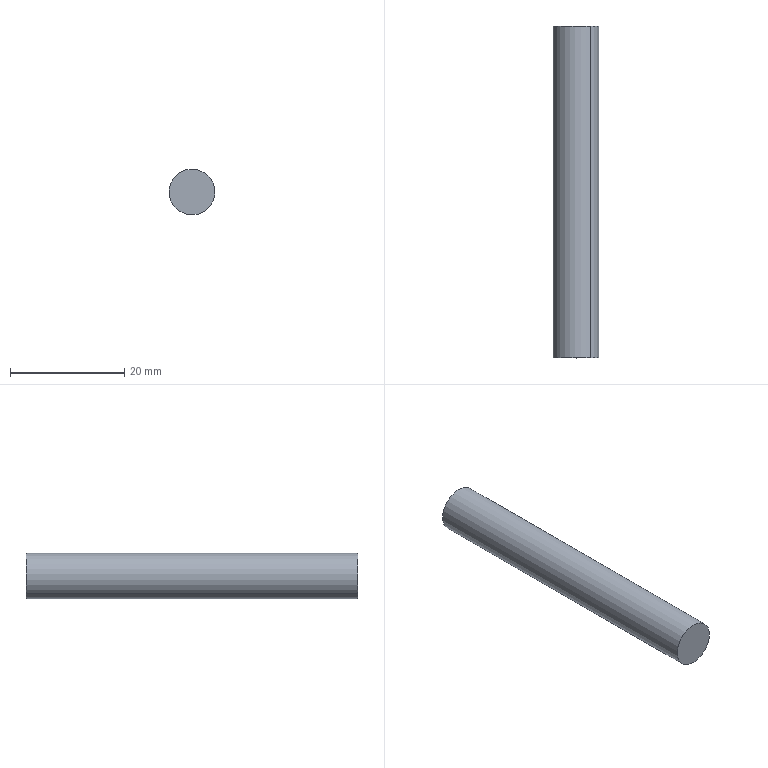Component | SolidWorks | DoorHinge3-1 | 1 solid | 4 faces | box 8 x 58 x 8 mm | volume 2915 mm3 | cylinder 2 | plane 2 | commonest cylinder face diameters 8 x2
build123d program:
from build123d import *

# Parameters (mm, degrees)
SKETCH1_R           = 4
BOSS_EXTRUDE1_DEPTH = 58


with BuildPart() as part:
    # Sketch1 → Boss-Extrude1 (new body)
    with BuildSketch(Plane(origin=(0, 0, 0), x_dir=(1, 0, 0), z_dir=(0, 1, 0))):
        with Locations(Location((0, 0, 0), (0, 0, 90))):
            Circle(SKETCH1_R)
    extrude(amount=BOSS_EXTRUDE1_DEPTH)


solid = part.part

# Placed as in the assembly
solid = solid.moved(Location((2175.473, 1880.46, 1245.107), (0, 0, 0)))
STEP:
#1=COLOUR_RGB('',0.7922,0.8196,0.9333);
#2=FILL_AREA_STYLE_COLOUR('',#1);
#3=FILL_AREA_STYLE('',(#2));
#4=SURFACE_STYLE_FILL_AREA(#3);
#5=SURFACE_SIDE_STYLE('',(#4));
#6=SURFACE_STYLE_USAGE(.BOTH.,#5);
#7=PRESENTATION_STYLE_ASSIGNMENT((#6));
#8=CARTESIAN_POINT('',(85.749,76.317,49.141));
#9=VERTEX_POINT('',#8);
#10=CARTESIAN_POINT('',(85.548,76.317,48.899));
#11=VERTEX_POINT('',#10);
#12=CARTESIAN_POINT('',(85.649,76.317,49.02));
#13=DIRECTION('',(-0.,1.,0.));
#14=DIRECTION('',(0.6365,0.,0.7713));
#15=AXIS2_PLACEMENT_3D('',#12,#13,#14);
#16=CIRCLE('',#15,0.1575);
#17=EDGE_CURVE('',#9,#11,#16,.T.);
#18=ORIENTED_EDGE('',*,*,#17,.F.);
#19=CARTESIAN_POINT('',(85.749,74.034,49.141));
#20=VERTEX_POINT('',#19);
#21=CARTESIAN_POINT('',(85.749,76.317,49.141));
#22=DIRECTION('',(0.,-1.,0.));
#23=VECTOR('',#22,39.37);
#24=LINE('',#21,#23);
#25=EDGE_CURVE('',#9,#20,#24,.T.);
#26=ORIENTED_EDGE('',*,*,#25,.T.);
#27=CARTESIAN_POINT('',(85.548,74.034,48.899));
#28=VERTEX_POINT('',#27);
#29=CARTESIAN_POINT('',(85.649,74.034,49.02));
#30=DIRECTION('',(-0.,1.,0.));
#31=DIRECTION('',(0.6365,0.,0.7713));
#32=AXIS2_PLACEMENT_3D('',#29,#30,#31);
#33=CIRCLE('',#32,0.1575);
#34=EDGE_CURVE('',#20,#28,#33,.T.);
#35=ORIENTED_EDGE('',*,*,#34,.T.);
#36=CARTESIAN_POINT('',(85.548,76.317,48.899));
#37=DIRECTION('',(0.,-1.,0.));
#38=VECTOR('',#37,39.37);
#39=LINE('',#36,#38);
#40=EDGE_CURVE('',#11,#28,#39,.T.);
#41=ORIENTED_EDGE('',*,*,#40,.F.);
#42=EDGE_LOOP('',(#18,#26,#35,#41));
#43=FACE_OUTER_BOUND('',#42,.T.);
#44=CARTESIAN_POINT('',(85.649,76.317,49.02));
#45=DIRECTION('',(0.,-1.,0.));
#46=DIRECTION('',(-0.6365,0.,-0.7713));
#47=AXIS2_PLACEMENT_3D('',#44,#45,#46);
#48=CYLINDRICAL_SURFACE('',#47,0.1575);
#49=ADVANCED_FACE('',(#43),#48,.T.);
#50=ORIENTED_EDGE('',*,*,#25,.F.);
#51=CARTESIAN_POINT('',(85.649,76.317,49.02));
#52=DIRECTION('',(-0.,1.,0.));
#53=DIRECTION('',(0.6365,0.,0.7713));
#54=AXIS2_PLACEMENT_3D('',#51,#52,#53);
#55=CIRCLE('',#54,0.1575);
#56=EDGE_CURVE('',#11,#9,#55,.T.);
#57=ORIENTED_EDGE('',*,*,#56,.F.);
#58=ORIENTED_EDGE('',*,*,#40,.T.);
#59=CARTESIAN_POINT('',(85.649,74.034,49.02));
#60=DIRECTION('',(-0.,1.,0.));
#61=DIRECTION('',(0.6365,0.,0.7713));
#62=AXIS2_PLACEMENT_3D('',#59,#60,#61);
#63=CIRCLE('',#62,0.1575);
#64=EDGE_CURVE('',#28,#20,#63,.T.);
#65=ORIENTED_EDGE('',*,*,#64,.T.);
#66=EDGE_LOOP('',(#50,#57,#58,#65));
#67=FACE_OUTER_BOUND('',#66,.T.);
#68=CARTESIAN_POINT('',(85.649,76.317,49.02));
#69=DIRECTION('',(0.,-1.,0.));
#70=DIRECTION('',(-0.6365,0.,-0.7713));
#71=AXIS2_PLACEMENT_3D('',#68,#69,#70);
#72=CYLINDRICAL_SURFACE('',#71,0.1575);
#73=ADVANCED_FACE('',(#67),#72,.T.);
#74=ORIENTED_EDGE('',*,*,#56,.T.);
#75=ORIENTED_EDGE('',*,*,#17,.T.);
#76=EDGE_LOOP('',(#74,#75));
#77=FACE_OUTER_BOUND('',#76,.T.);
#78=CARTESIAN_POINT('',(85.649,76.317,49.02));
#79=DIRECTION('',(-0.,1.,-0.));
#80=DIRECTION('',(0.6365,0.,0.7713));
#81=AXIS2_PLACEMENT_3D('',#78,#79,#80);
#82=PLANE('',#81);
#83=ADVANCED_FACE('',(#77),#82,.T.);
#84=ORIENTED_EDGE('',*,*,#64,.F.);
#85=ORIENTED_EDGE('',*,*,#34,.F.);
#86=EDGE_LOOP('',(#84,#85));
#87=FACE_OUTER_BOUND('',#86,.T.);
#88=CARTESIAN_POINT('',(85.649,74.034,49.02));
#89=DIRECTION('',(-0.,1.,-0.));
#90=DIRECTION('',(0.6365,0.,0.7713));
#91=AXIS2_PLACEMENT_3D('',#88,#89,#90);
#92=PLANE('',#91);
#93=ADVANCED_FACE('',(#87),#92,.F.);
#94=CLOSED_SHELL('',(#49,#73,#83,#93));
#95=MANIFOLD_SOLID_BREP('',#94);
#96=STYLED_ITEM('',(#7),#95);
#97=PRESENTATION_LAYER_ASSIGNMENT('','',(#96));
#98=(LENGTH_UNIT()NAMED_UNIT(*)SI_UNIT($,.METRE.));
#99=LENGTH_MEASURE_WITH_UNIT(LENGTH_MEASURE(0.0254),#98);
#100=DIMENSIONAL_EXPONENTS(1.,0.,0.,0.,0.,0.,0.);
#101=(CONVERSION_BASED_UNIT('',#99)LENGTH_UNIT()NAMED_UNIT(#100));
#102=UNCERTAINTY_MEASURE_WITH_UNIT(LENGTH_MEASURE(0.00001),#101,'','');
#103=(NAMED_UNIT(*)PLANE_ANGLE_UNIT()SI_UNIT($,.RADIAN.));
#104=(NAMED_UNIT(*)SI_UNIT($,.STERADIAN.)SOLID_ANGLE_UNIT());
#105=(GEOMETRIC_REPRESENTATION_CONTEXT(3)GLOBAL_UNCERTAINTY_ASSIGNED_CONTEXT((#102))GLOBAL_UNIT_ASSIGNED_CONTEXT((#101,#103,#104))REPRESENTATION_CONTEXT('',''));
#106=MECHANICAL_DESIGN_GEOMETRIC_PRESENTATION_REPRESENTATION('',(#96),#105);
#107=CARTESIAN_POINT('',(0.,0.,0.));
#108=DIRECTION('',(0.,0.,1.));
#109=DIRECTION('',(1.,0.,0.));
#110=AXIS2_PLACEMENT_3D('',#107,#108,#109);
#111=(LENGTH_UNIT()NAMED_UNIT(*)SI_UNIT($,.METRE.));
#112=LENGTH_MEASURE_WITH_UNIT(LENGTH_MEASURE(0.0254),#111);
#113=DIMENSIONAL_EXPONENTS(1.,0.,0.,0.,0.,0.,0.);
#114=(CONVERSION_BASED_UNIT('',#112)LENGTH_UNIT()NAMED_UNIT(#113));
#115=UNCERTAINTY_MEASURE_WITH_UNIT(LENGTH_MEASURE(0.00001),#114,'','');
#116=(NAMED_UNIT(*)PLANE_ANGLE_UNIT()SI_UNIT($,.RADIAN.));
#117=(NAMED_UNIT(*)SI_UNIT($,.STERADIAN.)SOLID_ANGLE_UNIT());
#118=(GEOMETRIC_REPRESENTATION_CONTEXT(3)GLOBAL_UNCERTAINTY_ASSIGNED_CONTEXT((#115))GLOBAL_UNIT_ASSIGNED_CONTEXT((#114,#116,#117))REPRESENTATION_CONTEXT('',''));
#119=ADVANCED_BREP_SHAPE_REPRESENTATION('',(#95,#110),#118);